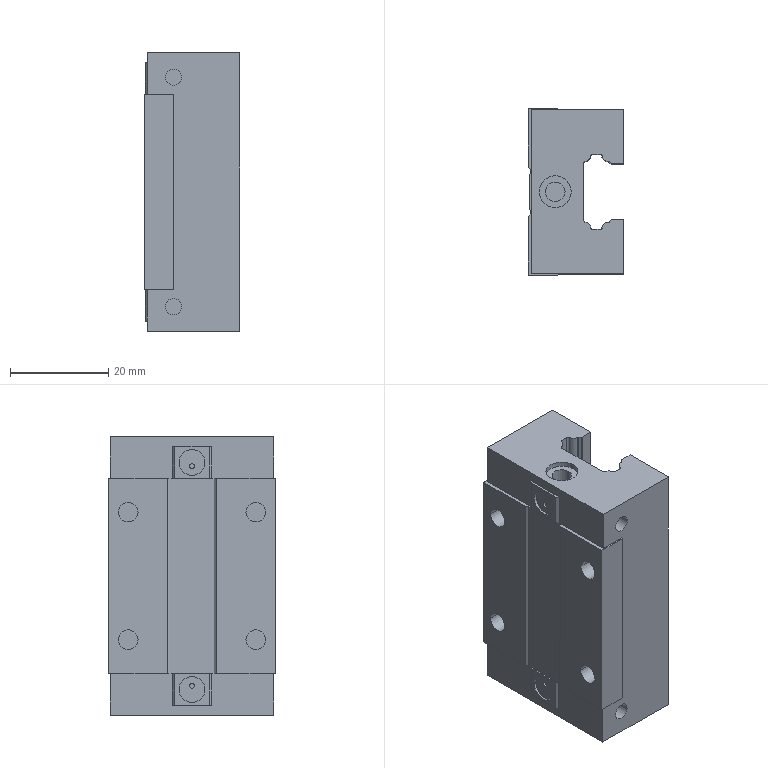Component | SolidWorks | 15LinearRailSlider-1 | 1 solid | 100 faces | box 19.55 x 34 x 56.82 mm | volume 29888 mm3 | plane 54 | cylinder 46 | commonest cylinder face diameters 4 x12 3.35 x8 0.96 x8 1 x4 5.3 x4 6.5 x4 2.5 x4 0.24 x2